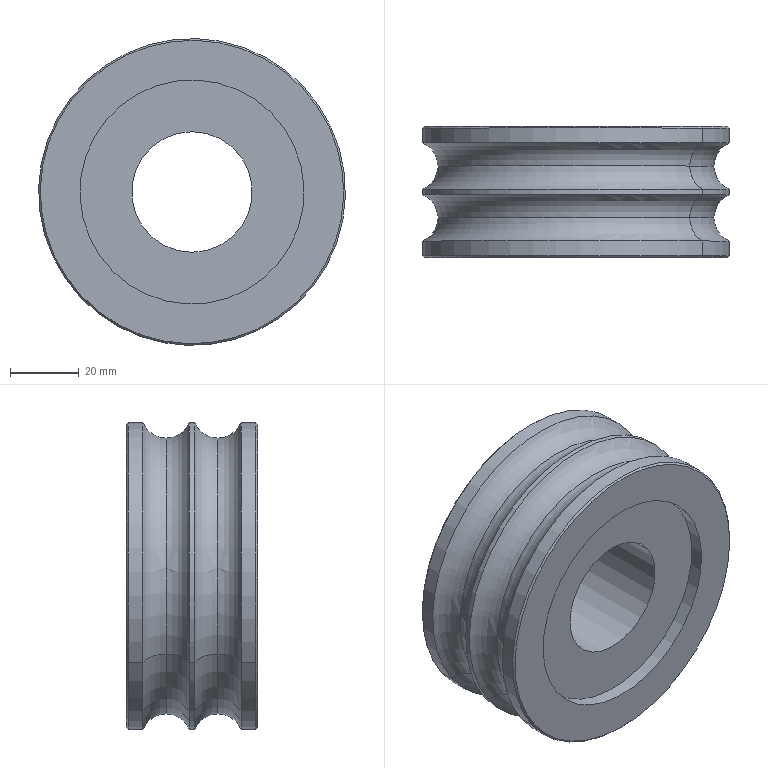Component | SolidWorks | 12ATransverseStraighteningPlatePart-2_12AStraighteningGrooveWheel-23_12ADoubleGrooveWheel-1 | 1 solid | 28 faces | box 89 x 38 x 89 mm | volume 157400 mm3 | cylinder 12 | torus 8 | cone 4 | plane 4 | commonest cylinder face diameters 89 x6 65 x4 35 x2 | material GCr15
build123d program:
from build123d import *

# Parameters (mm, degrees)
CHAMFER1_SIZE = 0.5
CHAMFER2_SIZE = 0.5


with BuildPart() as part:
    # Sketch1 → Revolve1 (revolve)
    with BuildSketch(Plane.XY, mode=Mode.PRIVATE) as revolve1_sk:
        with BuildLine():
            Line((0, 32.5), (0, 44.5))
            Line((0, 44.5), (4.75, 44.5))
            ThreePointArc((4.75, 44.5), (11.5, 40), (18.25, 44.5))
            Line((18.25, 44.5), (19.75, 44.5))
            ThreePointArc((19.75, 44.5), (26.5, 40), (33.25, 44.5))
            Line((33.25, 44.5), (38, 44.5))
            Line((38, 44.5), (38, 32.5))
            Line((38, 32.5), (34, 32.5))
            Line((34, 32.5), (34, 17.5))
            Line((34, 17.5), (4, 17.5))
            Line((4, 17.5), (4, 32.5))
            Line((4, 32.5), (0, 32.5))
        make_face()
    revolve(revolve1_sk.sketch.rotate(Axis((0, 0, 0), (1, 0, 0)), 180), axis=Axis((0, 0, 0), (1, 0, 0)))

    # Chamfer1
    chamfer1_edges = [part.edges().sort_by_distance(p)[0] for p in [
        (0, 44.5, 0),
    ]]
    chamfer(chamfer1_edges, length=CHAMFER1_SIZE)

    # Chamfer2
    chamfer2_edges = [part.edges().sort_by_distance(p)[0] for p in [
        (38, 44.5, 0),
    ]]
    chamfer(chamfer2_edges, length=CHAMFER2_SIZE)


solid = part.part

# Placed as in the assembly
solid = solid.moved(Location((206.117, 85.96, 213), (0, 0, 90)))
STEP:
#1=COLOUR_RGB('',0.7922,0.8196,0.9333);
#2=FILL_AREA_STYLE_COLOUR('',#1);
#3=FILL_AREA_STYLE('',(#2));
#4=SURFACE_STYLE_FILL_AREA(#3);
#5=SURFACE_SIDE_STYLE('',(#4));
#6=SURFACE_STYLE_USAGE(.BOTH.,#5);
#7=PRESENTATION_STYLE_ASSIGNMENT((#6));
#8=CARTESIAN_POINT('',(9.56,4.693,9.376));
#9=VERTEX_POINT('',#8);
#10=CARTESIAN_POINT('',(9.414,4.428,9.276));
#11=VERTEX_POINT('',#10);
#12=CARTESIAN_POINT('',(9.651,4.428,9.439));
#13=DIRECTION('',(-0.5653,-0.,0.8249));
#14=DIRECTION('',(0.8249,0.,0.5653));
#15=AXIS2_PLACEMENT_3D('',#12,#13,#14);
#16=CIRCLE('',#15,0.2879);
#17=EDGE_CURVE('',#9,#11,#16,.T.);
#18=ORIENTED_EDGE('',*,*,#17,.T.);
#19=CARTESIAN_POINT('',(6.816,4.428,7.496));
#20=VERTEX_POINT('',#19);
#21=CARTESIAN_POINT('',(8.115,4.428,8.386));
#22=DIRECTION('',(-0.,1.,0.));
#23=DIRECTION('',(-1.,-0.,0.));
#24=AXIS2_PLACEMENT_3D('',#21,#22,#23);
#25=CIRCLE('',#24,1.575);
#26=EDGE_CURVE('',#11,#20,#25,.T.);
#27=ORIENTED_EDGE('',*,*,#26,.T.);
#28=CARTESIAN_POINT('',(6.67,4.693,7.395));
#29=VERTEX_POINT('',#28);
#30=CARTESIAN_POINT('',(6.578,4.428,7.333));
#31=DIRECTION('',(0.5653,0.,-0.8249));
#32=DIRECTION('',(-0.8249,0.,-0.5653));
#33=AXIS2_PLACEMENT_3D('',#30,#31,#32);
#34=CIRCLE('',#33,0.2879);
#35=EDGE_CURVE('',#29,#20,#34,.T.);
#36=ORIENTED_EDGE('',*,*,#35,.F.);
#37=CARTESIAN_POINT('',(8.115,4.693,8.386));
#38=DIRECTION('',(-0.,1.,0.));
#39=DIRECTION('',(0.8249,0.,0.5653));
#40=AXIS2_PLACEMENT_3D('',#37,#38,#39);
#41=CIRCLE('',#40,1.752);
#42=EDGE_CURVE('',#9,#29,#41,.T.);
#43=ORIENTED_EDGE('',*,*,#42,.F.);
#44=EDGE_LOOP('',(#18,#27,#36,#43));
#45=FACE_OUTER_BOUND('',#44,.T.);
#46=CARTESIAN_POINT('',(8.115,4.428,8.386));
#47=DIRECTION('',(-0.,1.,0.));
#48=DIRECTION('',(0.8249,0.,0.5653));
#49=AXIS2_PLACEMENT_3D('',#46,#47,#48);
#50=TOROIDAL_SURFACE('',#49,1.863,0.2879);
#51=ADVANCED_FACE('',(#45),#50,.F.);
#52=CARTESIAN_POINT('',(9.56,4.103,9.376));
#53=VERTEX_POINT('',#52);
#54=CARTESIAN_POINT('',(9.414,3.837,9.276));
#55=VERTEX_POINT('',#54);
#56=CARTESIAN_POINT('',(9.651,3.837,9.439));
#57=DIRECTION('',(-0.5653,-0.,0.8249));
#58=DIRECTION('',(0.8249,0.,0.5653));
#59=AXIS2_PLACEMENT_3D('',#56,#57,#58);
#60=CIRCLE('',#59,0.2879);
#61=EDGE_CURVE('',#53,#55,#60,.T.);
#62=ORIENTED_EDGE('',*,*,#61,.T.);
#63=CARTESIAN_POINT('',(6.816,3.837,7.496));
#64=VERTEX_POINT('',#63);
#65=CARTESIAN_POINT('',(8.115,3.837,8.386));
#66=DIRECTION('',(-0.,1.,0.));
#67=DIRECTION('',(-1.,-0.,0.));
#68=AXIS2_PLACEMENT_3D('',#65,#66,#67);
#69=CIRCLE('',#68,1.575);
#70=EDGE_CURVE('',#55,#64,#69,.T.);
#71=ORIENTED_EDGE('',*,*,#70,.T.);
#72=CARTESIAN_POINT('',(6.67,4.103,7.395));
#73=VERTEX_POINT('',#72);
#74=CARTESIAN_POINT('',(6.578,3.837,7.333));
#75=DIRECTION('',(0.5653,0.,-0.8249));
#76=DIRECTION('',(-0.8249,0.,-0.5653));
#77=AXIS2_PLACEMENT_3D('',#74,#75,#76);
#78=CIRCLE('',#77,0.2879);
#79=EDGE_CURVE('',#73,#64,#78,.T.);
#80=ORIENTED_EDGE('',*,*,#79,.F.);
#81=CARTESIAN_POINT('',(8.115,4.103,8.386));
#82=DIRECTION('',(-0.,1.,0.));
#83=DIRECTION('',(0.8249,0.,0.5653));
#84=AXIS2_PLACEMENT_3D('',#81,#82,#83);
#85=CIRCLE('',#84,1.752);
#86=EDGE_CURVE('',#53,#73,#85,.T.);
#87=ORIENTED_EDGE('',*,*,#86,.F.);
#88=EDGE_LOOP('',(#62,#71,#80,#87));
#89=FACE_OUTER_BOUND('',#88,.T.);
#90=CARTESIAN_POINT('',(8.115,3.837,8.386));
#91=DIRECTION('',(-0.,1.,0.));
#92=DIRECTION('',(0.8249,0.,0.5653));
#93=AXIS2_PLACEMENT_3D('',#90,#91,#92);
#94=TOROIDAL_SURFACE('',#93,1.863,0.2879);
#95=ADVANCED_FACE('',(#89),#94,.F.);
#96=ORIENTED_EDGE('',*,*,#79,.T.);
#97=CARTESIAN_POINT('',(8.115,3.837,8.386));
#98=DIRECTION('',(-0.,1.,0.));
#99=DIRECTION('',(-1.,-0.,0.));
#100=AXIS2_PLACEMENT_3D('',#97,#98,#99);
#101=CIRCLE('',#100,1.575);
#102=EDGE_CURVE('',#64,#55,#101,.T.);
#103=ORIENTED_EDGE('',*,*,#102,.T.);
#104=ORIENTED_EDGE('',*,*,#61,.F.);
#105=CARTESIAN_POINT('',(8.115,4.103,8.386));
#106=DIRECTION('',(-0.,1.,0.));
#107=DIRECTION('',(0.8249,0.,0.5653));
#108=AXIS2_PLACEMENT_3D('',#105,#106,#107);
#109=CIRCLE('',#108,1.752);
#110=EDGE_CURVE('',#73,#53,#109,.T.);
#111=ORIENTED_EDGE('',*,*,#110,.F.);
#112=EDGE_LOOP('',(#96,#103,#104,#111));
#113=FACE_OUTER_BOUND('',#112,.T.);
#114=CARTESIAN_POINT('',(8.115,3.837,8.386));
#115=DIRECTION('',(-0.,1.,0.));
#116=DIRECTION('',(0.8249,0.,0.5653));
#117=AXIS2_PLACEMENT_3D('',#114,#115,#116);
#118=TOROIDAL_SURFACE('',#117,1.863,0.2879);
#119=ADVANCED_FACE('',(#113),#118,.F.);
#120=ORIENTED_EDGE('',*,*,#35,.T.);
#121=CARTESIAN_POINT('',(8.115,4.428,8.386));
#122=DIRECTION('',(-0.,1.,0.));
#123=DIRECTION('',(-1.,-0.,0.));
#124=AXIS2_PLACEMENT_3D('',#121,#122,#123);
#125=CIRCLE('',#124,1.575);
#126=EDGE_CURVE('',#20,#11,#125,.T.);
#127=ORIENTED_EDGE('',*,*,#126,.T.);
#128=ORIENTED_EDGE('',*,*,#17,.F.);
#129=CARTESIAN_POINT('',(8.115,4.693,8.386));
#130=DIRECTION('',(-0.,1.,0.));
#131=DIRECTION('',(0.8249,0.,0.5653));
#132=AXIS2_PLACEMENT_3D('',#129,#130,#131);
#133=CIRCLE('',#132,1.752);
#134=EDGE_CURVE('',#29,#9,#133,.T.);
#135=ORIENTED_EDGE('',*,*,#134,.F.);
#136=EDGE_LOOP('',(#120,#127,#128,#135));
#137=FACE_OUTER_BOUND('',#136,.T.);
#138=CARTESIAN_POINT('',(8.115,4.428,8.386));
#139=DIRECTION('',(-0.,1.,0.));
#140=DIRECTION('',(0.8249,0.,0.5653));
#141=AXIS2_PLACEMENT_3D('',#138,#139,#140);
#142=TOROIDAL_SURFACE('',#141,1.863,0.2879);
#143=ADVANCED_FACE('',(#137),#142,.F.);
#144=CARTESIAN_POINT('',(6.686,3.384,7.407));
#145=VERTEX_POINT('',#144);
#146=CARTESIAN_POINT('',(9.544,3.384,9.365));
#147=VERTEX_POINT('',#146);
#148=CARTESIAN_POINT('',(8.115,3.384,8.386));
#149=DIRECTION('',(0.,-1.,-0.));
#150=DIRECTION('',(0.8249,0.,0.5653));
#151=AXIS2_PLACEMENT_3D('',#148,#149,#150);
#152=CIRCLE('',#151,1.732);
#153=EDGE_CURVE('',#145,#147,#152,.T.);
#154=ORIENTED_EDGE('',*,*,#153,.F.);
#155=CARTESIAN_POINT('',(6.67,3.404,7.395));
#156=VERTEX_POINT('',#155);
#157=CARTESIAN_POINT('',(6.67,3.404,7.395));
#158=DIRECTION('',(-0.5833,0.7071,-0.3997));
#159=VECTOR('',#158,39.37);
#160=LINE('',#157,#159);
#161=EDGE_CURVE('',#145,#156,#160,.T.);
#162=ORIENTED_EDGE('',*,*,#161,.T.);
#163=CARTESIAN_POINT('',(9.56,3.404,9.376));
#164=VERTEX_POINT('',#163);
#165=CARTESIAN_POINT('',(8.115,3.404,8.386));
#166=DIRECTION('',(-0.,1.,0.));
#167=DIRECTION('',(0.8249,0.,0.5653));
#168=AXIS2_PLACEMENT_3D('',#165,#166,#167);
#169=CIRCLE('',#168,1.752);
#170=EDGE_CURVE('',#164,#156,#169,.T.);
#171=ORIENTED_EDGE('',*,*,#170,.F.);
#172=CARTESIAN_POINT('',(9.56,3.404,9.376));
#173=DIRECTION('',(0.5833,0.7071,0.3997));
#174=VECTOR('',#173,39.37);
#175=LINE('',#172,#174);
#176=EDGE_CURVE('',#147,#164,#175,.T.);
#177=ORIENTED_EDGE('',*,*,#176,.F.);
#178=EDGE_LOOP('',(#154,#162,#171,#177));
#179=FACE_OUTER_BOUND('',#178,.T.);
#180=CARTESIAN_POINT('',(8.115,3.404,8.386));
#181=DIRECTION('',(-0.,1.,0.));
#182=DIRECTION('',(0.8249,0.,0.5653));
#183=AXIS2_PLACEMENT_3D('',#180,#181,#182);
#184=CONICAL_SURFACE('',#183,1.752,0.7854);
#185=ADVANCED_FACE('',(#179),#184,.T.);
#186=CARTESIAN_POINT('',(9.544,4.88,9.365));
#187=VERTEX_POINT('',#186);
#188=CARTESIAN_POINT('',(6.686,4.88,7.407));
#189=VERTEX_POINT('',#188);
#190=CARTESIAN_POINT('',(8.115,4.88,8.386));
#191=DIRECTION('',(-0.,1.,0.));
#192=DIRECTION('',(-0.8249,-0.,-0.5653));
#193=AXIS2_PLACEMENT_3D('',#190,#191,#192);
#194=CIRCLE('',#193,1.732);
#195=EDGE_CURVE('',#187,#189,#194,.T.);
#196=ORIENTED_EDGE('',*,*,#195,.F.);
#197=CARTESIAN_POINT('',(9.56,4.861,9.376));
#198=VERTEX_POINT('',#197);
#199=CARTESIAN_POINT('',(9.544,4.88,9.365));
#200=DIRECTION('',(0.5833,-0.7071,0.3997));
#201=VECTOR('',#200,39.37);
#202=LINE('',#199,#201);
#203=EDGE_CURVE('',#187,#198,#202,.T.);
#204=ORIENTED_EDGE('',*,*,#203,.T.);
#205=CARTESIAN_POINT('',(6.67,4.861,7.395));
#206=VERTEX_POINT('',#205);
#207=CARTESIAN_POINT('',(8.115,4.861,8.386));
#208=DIRECTION('',(0.,-1.,-0.));
#209=DIRECTION('',(-0.8249,-0.,-0.5653));
#210=AXIS2_PLACEMENT_3D('',#207,#208,#209);
#211=CIRCLE('',#210,1.752);
#212=EDGE_CURVE('',#206,#198,#211,.T.);
#213=ORIENTED_EDGE('',*,*,#212,.F.);
#214=CARTESIAN_POINT('',(6.686,4.88,7.407));
#215=DIRECTION('',(-0.5833,-0.7071,-0.3997));
#216=VECTOR('',#215,39.37);
#217=LINE('',#214,#216);
#218=EDGE_CURVE('',#189,#206,#217,.T.);
#219=ORIENTED_EDGE('',*,*,#218,.F.);
#220=EDGE_LOOP('',(#196,#204,#213,#219));
#221=FACE_OUTER_BOUND('',#220,.T.);
#222=CARTESIAN_POINT('',(8.115,4.88,8.386));
#223=DIRECTION('',(0.,-1.,-0.));
#224=DIRECTION('',(-0.8249,-0.,-0.5653));
#225=AXIS2_PLACEMENT_3D('',#222,#223,#224);
#226=CONICAL_SURFACE('',#225,1.732,0.7854);
#227=ADVANCED_FACE('',(#221),#226,.T.);
#228=CARTESIAN_POINT('',(7.059,4.723,7.663));
#229=VERTEX_POINT('',#228);
#230=CARTESIAN_POINT('',(9.17,4.723,9.109));
#231=VERTEX_POINT('',#230);
#232=CARTESIAN_POINT('',(8.115,4.723,8.386));
#233=DIRECTION('',(-0.,1.,0.));
#234=DIRECTION('',(0.8249,0.,0.5653));
#235=AXIS2_PLACEMENT_3D('',#232,#233,#234);
#236=CIRCLE('',#235,1.28);
#237=EDGE_CURVE('',#229,#231,#236,.T.);
#238=ORIENTED_EDGE('',*,*,#237,.F.);
#239=CARTESIAN_POINT('',(7.059,4.88,7.663));
#240=VERTEX_POINT('',#239);
#241=CARTESIAN_POINT('',(7.059,4.88,7.663));
#242=DIRECTION('',(-0.,1.,0.));
#243=VECTOR('',#242,39.37);
#244=LINE('',#241,#243);
#245=EDGE_CURVE('',#229,#240,#244,.T.);
#246=ORIENTED_EDGE('',*,*,#245,.T.);
#247=CARTESIAN_POINT('',(9.17,4.88,9.109));
#248=VERTEX_POINT('',#247);
#249=CARTESIAN_POINT('',(8.115,4.88,8.386));
#250=DIRECTION('',(-0.,1.,0.));
#251=DIRECTION('',(0.8249,0.,0.5653));
#252=AXIS2_PLACEMENT_3D('',#249,#250,#251);
#253=CIRCLE('',#252,1.28);
#254=EDGE_CURVE('',#240,#248,#253,.T.);
#255=ORIENTED_EDGE('',*,*,#254,.T.);
#256=CARTESIAN_POINT('',(9.17,4.88,9.109));
#257=DIRECTION('',(-0.,1.,0.));
#258=VECTOR('',#257,39.37);
#259=LINE('',#256,#258);
#260=EDGE_CURVE('',#231,#248,#259,.T.);
#261=ORIENTED_EDGE('',*,*,#260,.F.);
#262=EDGE_LOOP('',(#238,#246,#255,#261));
#263=FACE_OUTER_BOUND('',#262,.T.);
#264=CARTESIAN_POINT('',(8.115,4.88,8.386));
#265=DIRECTION('',(-0.,1.,0.));
#266=DIRECTION('',(0.8249,0.,0.5653));
#267=AXIS2_PLACEMENT_3D('',#264,#265,#266);
#268=CYLINDRICAL_SURFACE('',#267,1.28);
#269=ADVANCED_FACE('',(#263),#268,.F.);
#270=ORIENTED_EDGE('',*,*,#42,.T.);
#271=CARTESIAN_POINT('',(6.67,4.88,7.395));
#272=DIRECTION('',(-0.,1.,0.));
#273=VECTOR('',#272,39.37);
#274=LINE('',#271,#273);
#275=EDGE_CURVE('',#29,#206,#274,.T.);
#276=ORIENTED_EDGE('',*,*,#275,.T.);
#277=ORIENTED_EDGE('',*,*,#212,.T.);
#278=CARTESIAN_POINT('',(9.56,4.88,9.376));
#279=DIRECTION('',(-0.,1.,0.));
#280=VECTOR('',#279,39.37);
#281=LINE('',#278,#280);
#282=EDGE_CURVE('',#9,#198,#281,.T.);
#283=ORIENTED_EDGE('',*,*,#282,.F.);
#284=EDGE_LOOP('',(#270,#276,#277,#283));
#285=FACE_OUTER_BOUND('',#284,.T.);
#286=CARTESIAN_POINT('',(8.115,4.88,8.386));
#287=DIRECTION('',(-0.,1.,0.));
#288=DIRECTION('',(0.8249,0.,0.5653));
#289=AXIS2_PLACEMENT_3D('',#286,#287,#288);
#290=CYLINDRICAL_SURFACE('',#289,1.752);
#291=ADVANCED_FACE('',(#285),#290,.T.);
#292=ORIENTED_EDGE('',*,*,#126,.F.);
#293=CARTESIAN_POINT('',(6.67,4.162,7.395));
#294=VERTEX_POINT('',#293);
#295=CARTESIAN_POINT('',(6.578,4.428,7.333));
#296=DIRECTION('',(0.5653,0.,-0.8249));
#297=DIRECTION('',(-0.8249,0.,-0.5653));
#298=AXIS2_PLACEMENT_3D('',#295,#296,#297);
#299=CIRCLE('',#298,0.2879);
#300=EDGE_CURVE('',#20,#294,#299,.T.);
#301=ORIENTED_EDGE('',*,*,#300,.T.);
#302=CARTESIAN_POINT('',(9.56,4.162,9.376));
#303=VERTEX_POINT('',#302);
#304=CARTESIAN_POINT('',(8.115,4.162,8.386));
#305=DIRECTION('',(-0.,1.,0.));
#306=DIRECTION('',(0.8249,0.,0.5653));
#307=AXIS2_PLACEMENT_3D('',#304,#305,#306);
#308=CIRCLE('',#307,1.752);
#309=EDGE_CURVE('',#294,#303,#308,.T.);
#310=ORIENTED_EDGE('',*,*,#309,.T.);
#311=CARTESIAN_POINT('',(9.651,4.428,9.439));
#312=DIRECTION('',(-0.5653,-0.,0.8249));
#313=DIRECTION('',(0.8249,0.,0.5653));
#314=AXIS2_PLACEMENT_3D('',#311,#312,#313);
#315=CIRCLE('',#314,0.2879);
#316=EDGE_CURVE('',#11,#303,#315,.T.);
#317=ORIENTED_EDGE('',*,*,#316,.F.);
#318=EDGE_LOOP('',(#292,#301,#310,#317));
#319=FACE_OUTER_BOUND('',#318,.T.);
#320=CARTESIAN_POINT('',(8.115,4.428,8.386));
#321=DIRECTION('',(-0.,1.,0.));
#322=DIRECTION('',(0.8249,0.,0.5653));
#323=AXIS2_PLACEMENT_3D('',#320,#321,#322);
#324=TOROIDAL_SURFACE('',#323,1.863,0.2879);
#325=ADVANCED_FACE('',(#319),#324,.F.);
#326=ORIENTED_EDGE('',*,*,#86,.T.);
#327=CARTESIAN_POINT('',(6.67,4.88,7.395));
#328=DIRECTION('',(-0.,1.,0.));
#329=VECTOR('',#328,39.37);
#330=LINE('',#327,#329);
#331=EDGE_CURVE('',#73,#294,#330,.T.);
#332=ORIENTED_EDGE('',*,*,#331,.T.);
#333=CARTESIAN_POINT('',(8.115,4.162,8.386));
#334=DIRECTION('',(-0.,1.,0.));
#335=DIRECTION('',(0.8249,0.,0.5653));
#336=AXIS2_PLACEMENT_3D('',#333,#334,#335);
#337=CIRCLE('',#336,1.752);
#338=EDGE_CURVE('',#303,#294,#337,.T.);
#339=ORIENTED_EDGE('',*,*,#338,.F.);
#340=CARTESIAN_POINT('',(9.56,4.88,9.376));
#341=DIRECTION('',(-0.,1.,0.));
#342=VECTOR('',#341,39.37);
#343=LINE('',#340,#342);
#344=EDGE_CURVE('',#53,#303,#343,.T.);
#345=ORIENTED_EDGE('',*,*,#344,.F.);
#346=EDGE_LOOP('',(#326,#332,#339,#345));
#347=FACE_OUTER_BOUND('',#346,.T.);
#348=CARTESIAN_POINT('',(8.115,4.88,8.386));
#349=DIRECTION('',(-0.,1.,0.));
#350=DIRECTION('',(0.8249,0.,0.5653));
#351=AXIS2_PLACEMENT_3D('',#348,#349,#350);
#352=CYLINDRICAL_SURFACE('',#351,1.752);
#353=ADVANCED_FACE('',(#347),#352,.T.);
#354=ORIENTED_EDGE('',*,*,#102,.F.);
#355=CARTESIAN_POINT('',(6.67,3.571,7.395));
#356=VERTEX_POINT('',#355);
#357=CARTESIAN_POINT('',(6.578,3.837,7.333));
#358=DIRECTION('',(0.5653,0.,-0.8249));
#359=DIRECTION('',(-0.8249,0.,-0.5653));
#360=AXIS2_PLACEMENT_3D('',#357,#358,#359);
#361=CIRCLE('',#360,0.2879);
#362=EDGE_CURVE('',#64,#356,#361,.T.);
#363=ORIENTED_EDGE('',*,*,#362,.T.);
#364=CARTESIAN_POINT('',(9.56,3.571,9.376));
#365=VERTEX_POINT('',#364);
#366=CARTESIAN_POINT('',(8.115,3.571,8.386));
#367=DIRECTION('',(-0.,1.,0.));
#368=DIRECTION('',(0.8249,0.,0.5653));
#369=AXIS2_PLACEMENT_3D('',#366,#367,#368);
#370=CIRCLE('',#369,1.752);
#371=EDGE_CURVE('',#356,#365,#370,.T.);
#372=ORIENTED_EDGE('',*,*,#371,.T.);
#373=CARTESIAN_POINT('',(9.651,3.837,9.439));
#374=DIRECTION('',(-0.5653,-0.,0.8249));
#375=DIRECTION('',(0.8249,0.,0.5653));
#376=AXIS2_PLACEMENT_3D('',#373,#374,#375);
#377=CIRCLE('',#376,0.2879);
#378=EDGE_CURVE('',#55,#365,#377,.T.);
#379=ORIENTED_EDGE('',*,*,#378,.F.);
#380=EDGE_LOOP('',(#354,#363,#372,#379));
#381=FACE_OUTER_BOUND('',#380,.T.);
#382=CARTESIAN_POINT('',(8.115,3.837,8.386));
#383=DIRECTION('',(-0.,1.,0.));
#384=DIRECTION('',(0.8249,0.,0.5653));
#385=AXIS2_PLACEMENT_3D('',#382,#383,#384);
#386=TOROIDAL_SURFACE('',#385,1.863,0.2879);
#387=ADVANCED_FACE('',(#381),#386,.F.);
#388=ORIENTED_EDGE('',*,*,#170,.T.);
#389=CARTESIAN_POINT('',(6.67,4.88,7.395));
#390=DIRECTION('',(-0.,1.,0.));
#391=VECTOR('',#390,39.37);
#392=LINE('',#389,#391);
#393=EDGE_CURVE('',#156,#356,#392,.T.);
#394=ORIENTED_EDGE('',*,*,#393,.T.);
#395=CARTESIAN_POINT('',(8.115,3.571,8.386));
#396=DIRECTION('',(-0.,1.,0.));
#397=DIRECTION('',(0.8249,0.,0.5653));
#398=AXIS2_PLACEMENT_3D('',#395,#396,#397);
#399=CIRCLE('',#398,1.752);
#400=EDGE_CURVE('',#365,#356,#399,.T.);
#401=ORIENTED_EDGE('',*,*,#400,.F.);
#402=CARTESIAN_POINT('',(9.56,4.88,9.376));
#403=DIRECTION('',(-0.,1.,0.));
#404=VECTOR('',#403,39.37);
#405=LINE('',#402,#404);
#406=EDGE_CURVE('',#164,#365,#405,.T.);
#407=ORIENTED_EDGE('',*,*,#406,.F.);
#408=EDGE_LOOP('',(#388,#394,#401,#407));
#409=FACE_OUTER_BOUND('',#408,.T.);
#410=CARTESIAN_POINT('',(8.115,4.88,8.386));
#411=DIRECTION('',(-0.,1.,0.));
#412=DIRECTION('',(0.8249,0.,0.5653));
#413=AXIS2_PLACEMENT_3D('',#410,#411,#412);
#414=CYLINDRICAL_SURFACE('',#413,1.752);
#415=ADVANCED_FACE('',(#409),#414,.T.);
#416=CARTESIAN_POINT('',(7.059,3.384,7.663));
#417=VERTEX_POINT('',#416);
#418=CARTESIAN_POINT('',(9.17,3.384,9.109));
#419=VERTEX_POINT('',#418);
#420=CARTESIAN_POINT('',(8.115,3.384,8.386));
#421=DIRECTION('',(-0.,1.,0.));
#422=DIRECTION('',(0.8249,0.,0.5653));
#423=AXIS2_PLACEMENT_3D('',#420,#421,#422);
#424=CIRCLE('',#423,1.28);
#425=EDGE_CURVE('',#417,#419,#424,.T.);
#426=ORIENTED_EDGE('',*,*,#425,.F.);
#427=CARTESIAN_POINT('',(7.059,3.542,7.663));
#428=VERTEX_POINT('',#427);
#429=CARTESIAN_POINT('',(7.059,4.88,7.663));
#430=DIRECTION('',(-0.,1.,0.));
#431=VECTOR('',#430,39.37);
#432=LINE('',#429,#431);
#433=EDGE_CURVE('',#417,#428,#432,.T.);
#434=ORIENTED_EDGE('',*,*,#433,.T.);
#435=CARTESIAN_POINT('',(9.17,3.542,9.109));
#436=VERTEX_POINT('',#435);
#437=CARTESIAN_POINT('',(8.115,3.542,8.386));
#438=DIRECTION('',(-0.,1.,0.));
#439=DIRECTION('',(0.8249,0.,0.5653));
#440=AXIS2_PLACEMENT_3D('',#437,#438,#439);
#441=CIRCLE('',#440,1.28);
#442=EDGE_CURVE('',#428,#436,#441,.T.);
#443=ORIENTED_EDGE('',*,*,#442,.T.);
#444=CARTESIAN_POINT('',(9.17,4.88,9.109));
#445=DIRECTION('',(-0.,1.,0.));
#446=VECTOR('',#445,39.37);
#447=LINE('',#444,#446);
#448=EDGE_CURVE('',#419,#436,#447,.T.);
#449=ORIENTED_EDGE('',*,*,#448,.F.);
#450=EDGE_LOOP('',(#426,#434,#443,#449));
#451=FACE_OUTER_BOUND('',#450,.T.);
#452=CARTESIAN_POINT('',(8.115,4.88,8.386));
#453=DIRECTION('',(-0.,1.,0.));
#454=DIRECTION('',(0.8249,0.,0.5653));
#455=AXIS2_PLACEMENT_3D('',#452,#453,#454);
#456=CYLINDRICAL_SURFACE('',#455,1.28);
#457=ADVANCED_FACE('',(#451),#456,.F.);
#458=CARTESIAN_POINT('',(7.547,3.542,7.996));
#459=VERTEX_POINT('',#458);
#460=CARTESIAN_POINT('',(8.683,3.542,8.775));
#461=VERTEX_POINT('',#460);
#462=CARTESIAN_POINT('',(8.115,3.542,8.386));
#463=DIRECTION('',(-0.,1.,0.));
#464=DIRECTION('',(0.8249,0.,0.5653));
#465=AXIS2_PLACEMENT_3D('',#462,#463,#464);
#466=CIRCLE('',#465,0.689);
#467=EDGE_CURVE('',#459,#461,#466,.T.);
#468=ORIENTED_EDGE('',*,*,#467,.F.);
#469=CARTESIAN_POINT('',(7.547,4.723,7.996));
#470=VERTEX_POINT('',#469);
#471=CARTESIAN_POINT('',(7.547,4.88,7.996));
#472=DIRECTION('',(-0.,1.,0.));
#473=VECTOR('',#472,39.37);
#474=LINE('',#471,#473);
#475=EDGE_CURVE('',#459,#470,#474,.T.);
#476=ORIENTED_EDGE('',*,*,#475,.T.);
#477=CARTESIAN_POINT('',(8.683,4.723,8.775));
#478=VERTEX_POINT('',#477);
#479=CARTESIAN_POINT('',(8.115,4.723,8.386));
#480=DIRECTION('',(-0.,1.,0.));
#481=DIRECTION('',(0.8249,0.,0.5653));
#482=AXIS2_PLACEMENT_3D('',#479,#480,#481);
#483=CIRCLE('',#482,0.689);
#484=EDGE_CURVE('',#470,#478,#483,.T.);
#485=ORIENTED_EDGE('',*,*,#484,.T.);
#486=CARTESIAN_POINT('',(8.683,4.88,8.775));
#487=DIRECTION('',(-0.,1.,0.));
#488=VECTOR('',#487,39.37);
#489=LINE('',#486,#488);
#490=EDGE_CURVE('',#461,#478,#489,.T.);
#491=ORIENTED_EDGE('',*,*,#490,.F.);
#492=EDGE_LOOP('',(#468,#476,#485,#491));
#493=FACE_OUTER_BOUND('',#492,.T.);
#494=CARTESIAN_POINT('',(8.115,4.88,8.386));
#495=DIRECTION('',(-0.,1.,0.));
#496=DIRECTION('',(0.8249,0.,0.5653));
#497=AXIS2_PLACEMENT_3D('',#494,#495,#496);
#498=CYLINDRICAL_SURFACE('',#497,0.689);
#499=ADVANCED_FACE('',(#493),#498,.F.);
#500=CARTESIAN_POINT('',(8.115,4.723,8.386));
#501=DIRECTION('',(-0.,1.,0.));
#502=DIRECTION('',(0.8249,0.,0.5653));
#503=AXIS2_PLACEMENT_3D('',#500,#501,#502);
#504=CIRCLE('',#503,0.689);
#505=EDGE_CURVE('',#478,#470,#504,.T.);
#506=ORIENTED_EDGE('',*,*,#505,.F.);
#507=ORIENTED_EDGE('',*,*,#484,.F.);
#508=EDGE_LOOP('',(#506,#507));
#509=FACE_BOUND('',#508,.T.);
#510=CARTESIAN_POINT('',(8.115,4.723,8.386));
#511=DIRECTION('',(-0.,1.,0.));
#512=DIRECTION('',(0.8249,0.,0.5653));
#513=AXIS2_PLACEMENT_3D('',#510,#511,#512);
#514=CIRCLE('',#513,1.28);
#515=EDGE_CURVE('',#231,#229,#514,.T.);
#516=ORIENTED_EDGE('',*,*,#515,.T.);
#517=ORIENTED_EDGE('',*,*,#237,.T.);
#518=EDGE_LOOP('',(#516,#517));
#519=FACE_OUTER_BOUND('',#518,.T.);
#520=CARTESIAN_POINT('',(7.059,4.723,7.663));
#521=DIRECTION('',(0.,-1.,0.));
#522=DIRECTION('',(-0.8249,-0.,-0.5653));
#523=AXIS2_PLACEMENT_3D('',#520,#521,#522);
#524=PLANE('',#523);
#525=ADVANCED_FACE('',(#509,#519),#524,.F.);
#526=ORIENTED_EDGE('',*,*,#475,.F.);
#527=CARTESIAN_POINT('',(8.115,3.542,8.386));
#528=DIRECTION('',(-0.,1.,0.));
#529=DIRECTION('',(0.8249,0.,0.5653));
#530=AXIS2_PLACEMENT_3D('',#527,#528,#529);
#531=CIRCLE('',#530,0.689);
#532=EDGE_CURVE('',#461,#459,#531,.T.);
#533=ORIENTED_EDGE('',*,*,#532,.F.);
#534=ORIENTED_EDGE('',*,*,#490,.T.);
#535=ORIENTED_EDGE('',*,*,#505,.T.);
#536=EDGE_LOOP('',(#526,#533,#534,#535));
#537=FACE_OUTER_BOUND('',#536,.T.);
#538=CARTESIAN_POINT('',(8.115,4.88,8.386));
#539=DIRECTION('',(-0.,1.,0.));
#540=DIRECTION('',(0.8249,0.,0.5653));
#541=AXIS2_PLACEMENT_3D('',#538,#539,#540);
#542=CYLINDRICAL_SURFACE('',#541,0.689);
#543=ADVANCED_FACE('',(#537),#542,.F.);
#544=CARTESIAN_POINT('',(8.115,3.542,8.386));
#545=DIRECTION('',(-0.,1.,0.));
#546=DIRECTION('',(0.8249,0.,0.5653));
#547=AXIS2_PLACEMENT_3D('',#544,#545,#546);
#548=CIRCLE('',#547,1.28);
#549=EDGE_CURVE('',#436,#428,#548,.T.);
#550=ORIENTED_EDGE('',*,*,#549,.F.);
#551=ORIENTED_EDGE('',*,*,#442,.F.);
#552=EDGE_LOOP('',(#550,#551));
#553=FACE_OUTER_BOUND('',#552,.T.);
#554=ORIENTED_EDGE('',*,*,#532,.T.);
#555=ORIENTED_EDGE('',*,*,#467,.T.);
#556=EDGE_LOOP('',(#554,#555));
#557=FACE_BOUND('',#556,.T.);
#558=CARTESIAN_POINT('',(7.547,3.542,7.996));
#559=DIRECTION('',(-0.,1.,-0.));
#560=DIRECTION('',(0.8249,0.,0.5653));
#561=AXIS2_PLACEMENT_3D('',#558,#559,#560);
#562=PLANE('',#561);
#563=ADVANCED_FACE('',(#553,#557),#562,.F.);
#564=ORIENTED_EDGE('',*,*,#433,.F.);
#565=CARTESIAN_POINT('',(8.115,3.384,8.386));
#566=DIRECTION('',(-0.,1.,0.));
#567=DIRECTION('',(0.8249,0.,0.5653));
#568=AXIS2_PLACEMENT_3D('',#565,#566,#567);
#569=CIRCLE('',#568,1.28);
#570=EDGE_CURVE('',#419,#417,#569,.T.);
#571=ORIENTED_EDGE('',*,*,#570,.F.);
#572=ORIENTED_EDGE('',*,*,#448,.T.);
#573=ORIENTED_EDGE('',*,*,#549,.T.);
#574=EDGE_LOOP('',(#564,#571,#572,#573));
#575=FACE_OUTER_BOUND('',#574,.T.);
#576=CARTESIAN_POINT('',(8.115,4.88,8.386));
#577=DIRECTION('',(-0.,1.,0.));
#578=DIRECTION('',(0.8249,0.,0.5653));
#579=AXIS2_PLACEMENT_3D('',#576,#577,#578);
#580=CYLINDRICAL_SURFACE('',#579,1.28);
#581=ADVANCED_FACE('',(#575),#580,.F.);
#582=CARTESIAN_POINT('',(8.115,3.384,8.386));
#583=DIRECTION('',(0.,-1.,-0.));
#584=DIRECTION('',(0.8249,0.,0.5653));
#585=AXIS2_PLACEMENT_3D('',#582,#583,#584);
#586=CIRCLE('',#585,1.732);
#587=EDGE_CURVE('',#147,#145,#586,.T.);
#588=ORIENTED_EDGE('',*,*,#587,.T.);
#589=ORIENTED_EDGE('',*,*,#153,.T.);
#590=EDGE_LOOP('',(#588,#589));
#591=FACE_OUTER_BOUND('',#590,.T.);
#592=ORIENTED_EDGE('',*,*,#570,.T.);
#593=ORIENTED_EDGE('',*,*,#425,.T.);
#594=EDGE_LOOP('',(#592,#593));
#595=FACE_BOUND('',#594,.T.);
#596=CARTESIAN_POINT('',(6.67,3.384,7.395));
#597=DIRECTION('',(-0.,1.,-0.));
#598=DIRECTION('',(0.8249,0.,0.5653));
#599=AXIS2_PLACEMENT_3D('',#596,#597,#598);
#600=PLANE('',#599);
#601=ADVANCED_FACE('',(#591,#595),#600,.F.);
#602=ORIENTED_EDGE('',*,*,#393,.F.);
#603=CARTESIAN_POINT('',(8.115,3.404,8.386));
#604=DIRECTION('',(-0.,1.,0.));
#605=DIRECTION('',(0.8249,0.,0.5653));
#606=AXIS2_PLACEMENT_3D('',#603,#604,#605);
#607=CIRCLE('',#606,1.752);
#608=EDGE_CURVE('',#156,#164,#607,.T.);
#609=ORIENTED_EDGE('',*,*,#608,.T.);
#610=ORIENTED_EDGE('',*,*,#406,.T.);
#611=ORIENTED_EDGE('',*,*,#371,.F.);
#612=EDGE_LOOP('',(#602,#609,#610,#611));
#613=FACE_OUTER_BOUND('',#612,.T.);
#614=CARTESIAN_POINT('',(8.115,4.88,8.386));
#615=DIRECTION('',(-0.,1.,0.));
#616=DIRECTION('',(0.8249,0.,0.5653));
#617=AXIS2_PLACEMENT_3D('',#614,#615,#616);
#618=CYLINDRICAL_SURFACE('',#617,1.752);
#619=ADVANCED_FACE('',(#613),#618,.T.);
#620=ORIENTED_EDGE('',*,*,#70,.F.);
#621=ORIENTED_EDGE('',*,*,#378,.T.);
#622=ORIENTED_EDGE('',*,*,#400,.T.);
#623=ORIENTED_EDGE('',*,*,#362,.F.);
#624=EDGE_LOOP('',(#620,#621,#622,#623));
#625=FACE_OUTER_BOUND('',#624,.T.);
#626=CARTESIAN_POINT('',(8.115,3.837,8.386));
#627=DIRECTION('',(-0.,1.,0.));
#628=DIRECTION('',(0.8249,0.,0.5653));
#629=AXIS2_PLACEMENT_3D('',#626,#627,#628);
#630=TOROIDAL_SURFACE('',#629,1.863,0.2879);
#631=ADVANCED_FACE('',(#625),#630,.F.);
#632=ORIENTED_EDGE('',*,*,#331,.F.);
#633=ORIENTED_EDGE('',*,*,#110,.T.);
#634=ORIENTED_EDGE('',*,*,#344,.T.);
#635=ORIENTED_EDGE('',*,*,#309,.F.);
#636=EDGE_LOOP('',(#632,#633,#634,#635));
#637=FACE_OUTER_BOUND('',#636,.T.);
#638=CARTESIAN_POINT('',(8.115,4.88,8.386));
#639=DIRECTION('',(-0.,1.,0.));
#640=DIRECTION('',(0.8249,0.,0.5653));
#641=AXIS2_PLACEMENT_3D('',#638,#639,#640);
#642=CYLINDRICAL_SURFACE('',#641,1.752);
#643=ADVANCED_FACE('',(#637),#642,.T.);
#644=ORIENTED_EDGE('',*,*,#26,.F.);
#645=ORIENTED_EDGE('',*,*,#316,.T.);
#646=ORIENTED_EDGE('',*,*,#338,.T.);
#647=ORIENTED_EDGE('',*,*,#300,.F.);
#648=EDGE_LOOP('',(#644,#645,#646,#647));
#649=FACE_OUTER_BOUND('',#648,.T.);
#650=CARTESIAN_POINT('',(8.115,4.428,8.386));
#651=DIRECTION('',(-0.,1.,0.));
#652=DIRECTION('',(0.8249,0.,0.5653));
#653=AXIS2_PLACEMENT_3D('',#650,#651,#652);
#654=TOROIDAL_SURFACE('',#653,1.863,0.2879);
#655=ADVANCED_FACE('',(#649),#654,.F.);
#656=ORIENTED_EDGE('',*,*,#275,.F.);
#657=ORIENTED_EDGE('',*,*,#134,.T.);
#658=ORIENTED_EDGE('',*,*,#282,.T.);
#659=CARTESIAN_POINT('',(8.115,4.861,8.386));
#660=DIRECTION('',(0.,-1.,-0.));
#661=DIRECTION('',(-0.8249,-0.,-0.5653));
#662=AXIS2_PLACEMENT_3D('',#659,#660,#661);
#663=CIRCLE('',#662,1.752);
#664=EDGE_CURVE('',#198,#206,#663,.T.);
#665=ORIENTED_EDGE('',*,*,#664,.T.);
#666=EDGE_LOOP('',(#656,#657,#658,#665));
#667=FACE_OUTER_BOUND('',#666,.T.);
#668=CARTESIAN_POINT('',(8.115,4.88,8.386));
#669=DIRECTION('',(-0.,1.,0.));
#670=DIRECTION('',(0.8249,0.,0.5653));
#671=AXIS2_PLACEMENT_3D('',#668,#669,#670);
#672=CYLINDRICAL_SURFACE('',#671,1.752);
#673=ADVANCED_FACE('',(#667),#672,.T.);
#674=CARTESIAN_POINT('',(8.115,4.88,8.386));
#675=DIRECTION('',(-0.,1.,0.));
#676=DIRECTION('',(-0.8249,-0.,-0.5653));
#677=AXIS2_PLACEMENT_3D('',#674,#675,#676);
#678=CIRCLE('',#677,1.732);
#679=EDGE_CURVE('',#189,#187,#678,.T.);
#680=ORIENTED_EDGE('',*,*,#679,.T.);
#681=ORIENTED_EDGE('',*,*,#195,.T.);
#682=EDGE_LOOP('',(#680,#681));
#683=FACE_OUTER_BOUND('',#682,.T.);
#684=CARTESIAN_POINT('',(8.115,4.88,8.386));
#685=DIRECTION('',(-0.,1.,0.));
#686=DIRECTION('',(0.8249,0.,0.5653));
#687=AXIS2_PLACEMENT_3D('',#684,#685,#686);
#688=CIRCLE('',#687,1.28);
#689=EDGE_CURVE('',#248,#240,#688,.T.);
#690=ORIENTED_EDGE('',*,*,#689,.F.);
#691=ORIENTED_EDGE('',*,*,#254,.F.);
#692=EDGE_LOOP('',(#690,#691));
#693=FACE_BOUND('',#692,.T.);
#694=CARTESIAN_POINT('',(7.059,4.88,7.663));
#695=DIRECTION('',(0.,-1.,0.));
#696=DIRECTION('',(-0.8249,-0.,-0.5653));
#697=AXIS2_PLACEMENT_3D('',#694,#695,#696);
#698=PLANE('',#697);
#699=ADVANCED_FACE('',(#683,#693),#698,.F.);
#700=ORIENTED_EDGE('',*,*,#245,.F.);
#701=ORIENTED_EDGE('',*,*,#515,.F.);
#702=ORIENTED_EDGE('',*,*,#260,.T.);
#703=ORIENTED_EDGE('',*,*,#689,.T.);
#704=EDGE_LOOP('',(#700,#701,#702,#703));
#705=FACE_OUTER_BOUND('',#704,.T.);
#706=CARTESIAN_POINT('',(8.115,4.88,8.386));
#707=DIRECTION('',(-0.,1.,0.));
#708=DIRECTION('',(0.8249,0.,0.5653));
#709=AXIS2_PLACEMENT_3D('',#706,#707,#708);
#710=CYLINDRICAL_SURFACE('',#709,1.28);
#711=ADVANCED_FACE('',(#705),#710,.F.);
#712=ORIENTED_EDGE('',*,*,#203,.F.);
#713=ORIENTED_EDGE('',*,*,#679,.F.);
#714=ORIENTED_EDGE('',*,*,#218,.T.);
#715=ORIENTED_EDGE('',*,*,#664,.F.);
#716=EDGE_LOOP('',(#712,#713,#714,#715));
#717=FACE_OUTER_BOUND('',#716,.T.);
#718=CARTESIAN_POINT('',(8.115,4.88,8.386));
#719=DIRECTION('',(0.,-1.,-0.));
#720=DIRECTION('',(-0.8249,-0.,-0.5653));
#721=AXIS2_PLACEMENT_3D('',#718,#719,#720);
#722=CONICAL_SURFACE('',#721,1.732,0.7854);
#723=ADVANCED_FACE('',(#717),#722,.T.);
#724=ORIENTED_EDGE('',*,*,#161,.F.);
#725=ORIENTED_EDGE('',*,*,#587,.F.);
#726=ORIENTED_EDGE('',*,*,#176,.T.);
#727=ORIENTED_EDGE('',*,*,#608,.F.);
#728=EDGE_LOOP('',(#724,#725,#726,#727));
#729=FACE_OUTER_BOUND('',#728,.T.);
#730=CARTESIAN_POINT('',(8.115,3.404,8.386));
#731=DIRECTION('',(-0.,1.,0.));
#732=DIRECTION('',(0.8249,0.,0.5653));
#733=AXIS2_PLACEMENT_3D('',#730,#731,#732);
#734=CONICAL_SURFACE('',#733,1.752,0.7854);
#735=ADVANCED_FACE('',(#729),#734,.T.);
#736=CLOSED_SHELL('',(#51,#95,#119,#143,#185,#227,#269,#291,#325,#353,#387,#415,#457,#499,#525,#543,#563,#581,#601,#619,#631,#643,#655,#673,#699,#711,#723,#735));
#737=MANIFOLD_SOLID_BREP('',#736);
#738=STYLED_ITEM('',(#7),#737);
#739=(LENGTH_UNIT()NAMED_UNIT(*)SI_UNIT($,.METRE.));
#740=LENGTH_MEASURE_WITH_UNIT(LENGTH_MEASURE(0.0254),#739);
#741=DIMENSIONAL_EXPONENTS(1.,0.,0.,0.,0.,0.,0.);
#742=(CONVERSION_BASED_UNIT('',#740)LENGTH_UNIT()NAMED_UNIT(#741));
#743=UNCERTAINTY_MEASURE_WITH_UNIT(LENGTH_MEASURE(0.00001),#742,'','');
#744=(NAMED_UNIT(*)PLANE_ANGLE_UNIT()SI_UNIT($,.RADIAN.));
#745=(NAMED_UNIT(*)SI_UNIT($,.STERADIAN.)SOLID_ANGLE_UNIT());
#746=(GEOMETRIC_REPRESENTATION_CONTEXT(3)GLOBAL_UNCERTAINTY_ASSIGNED_CONTEXT((#743))GLOBAL_UNIT_ASSIGNED_CONTEXT((#742,#744,#745))REPRESENTATION_CONTEXT('',''));
#747=MECHANICAL_DESIGN_GEOMETRIC_PRESENTATION_REPRESENTATION('',(#738),#746);
#748=PRESENTATION_LAYER_ASSIGNMENT('','',(#738));
#749=CARTESIAN_POINT('',(0.,0.,0.));
#750=DIRECTION('',(0.,0.,1.));
#751=DIRECTION('',(1.,0.,0.));
#752=AXIS2_PLACEMENT_3D('',#749,#750,#751);
#753=(LENGTH_UNIT()NAMED_UNIT(*)SI_UNIT($,.METRE.));
#754=LENGTH_MEASURE_WITH_UNIT(LENGTH_MEASURE(0.0254),#753);
#755=DIMENSIONAL_EXPONENTS(1.,0.,0.,0.,0.,0.,0.);
#756=(CONVERSION_BASED_UNIT('',#754)LENGTH_UNIT()NAMED_UNIT(#755));
#757=UNCERTAINTY_MEASURE_WITH_UNIT(LENGTH_MEASURE(0.00001),#756,'','');
#758=(NAMED_UNIT(*)PLANE_ANGLE_UNIT()SI_UNIT($,.RADIAN.));
#759=(NAMED_UNIT(*)SI_UNIT($,.STERADIAN.)SOLID_ANGLE_UNIT());
#760=(GEOMETRIC_REPRESENTATION_CONTEXT(3)GLOBAL_UNCERTAINTY_ASSIGNED_CONTEXT((#757))GLOBAL_UNIT_ASSIGNED_CONTEXT((#756,#758,#759))REPRESENTATION_CONTEXT('',''));
#761=ADVANCED_BREP_SHAPE_REPRESENTATION('',(#737,#752),#760);